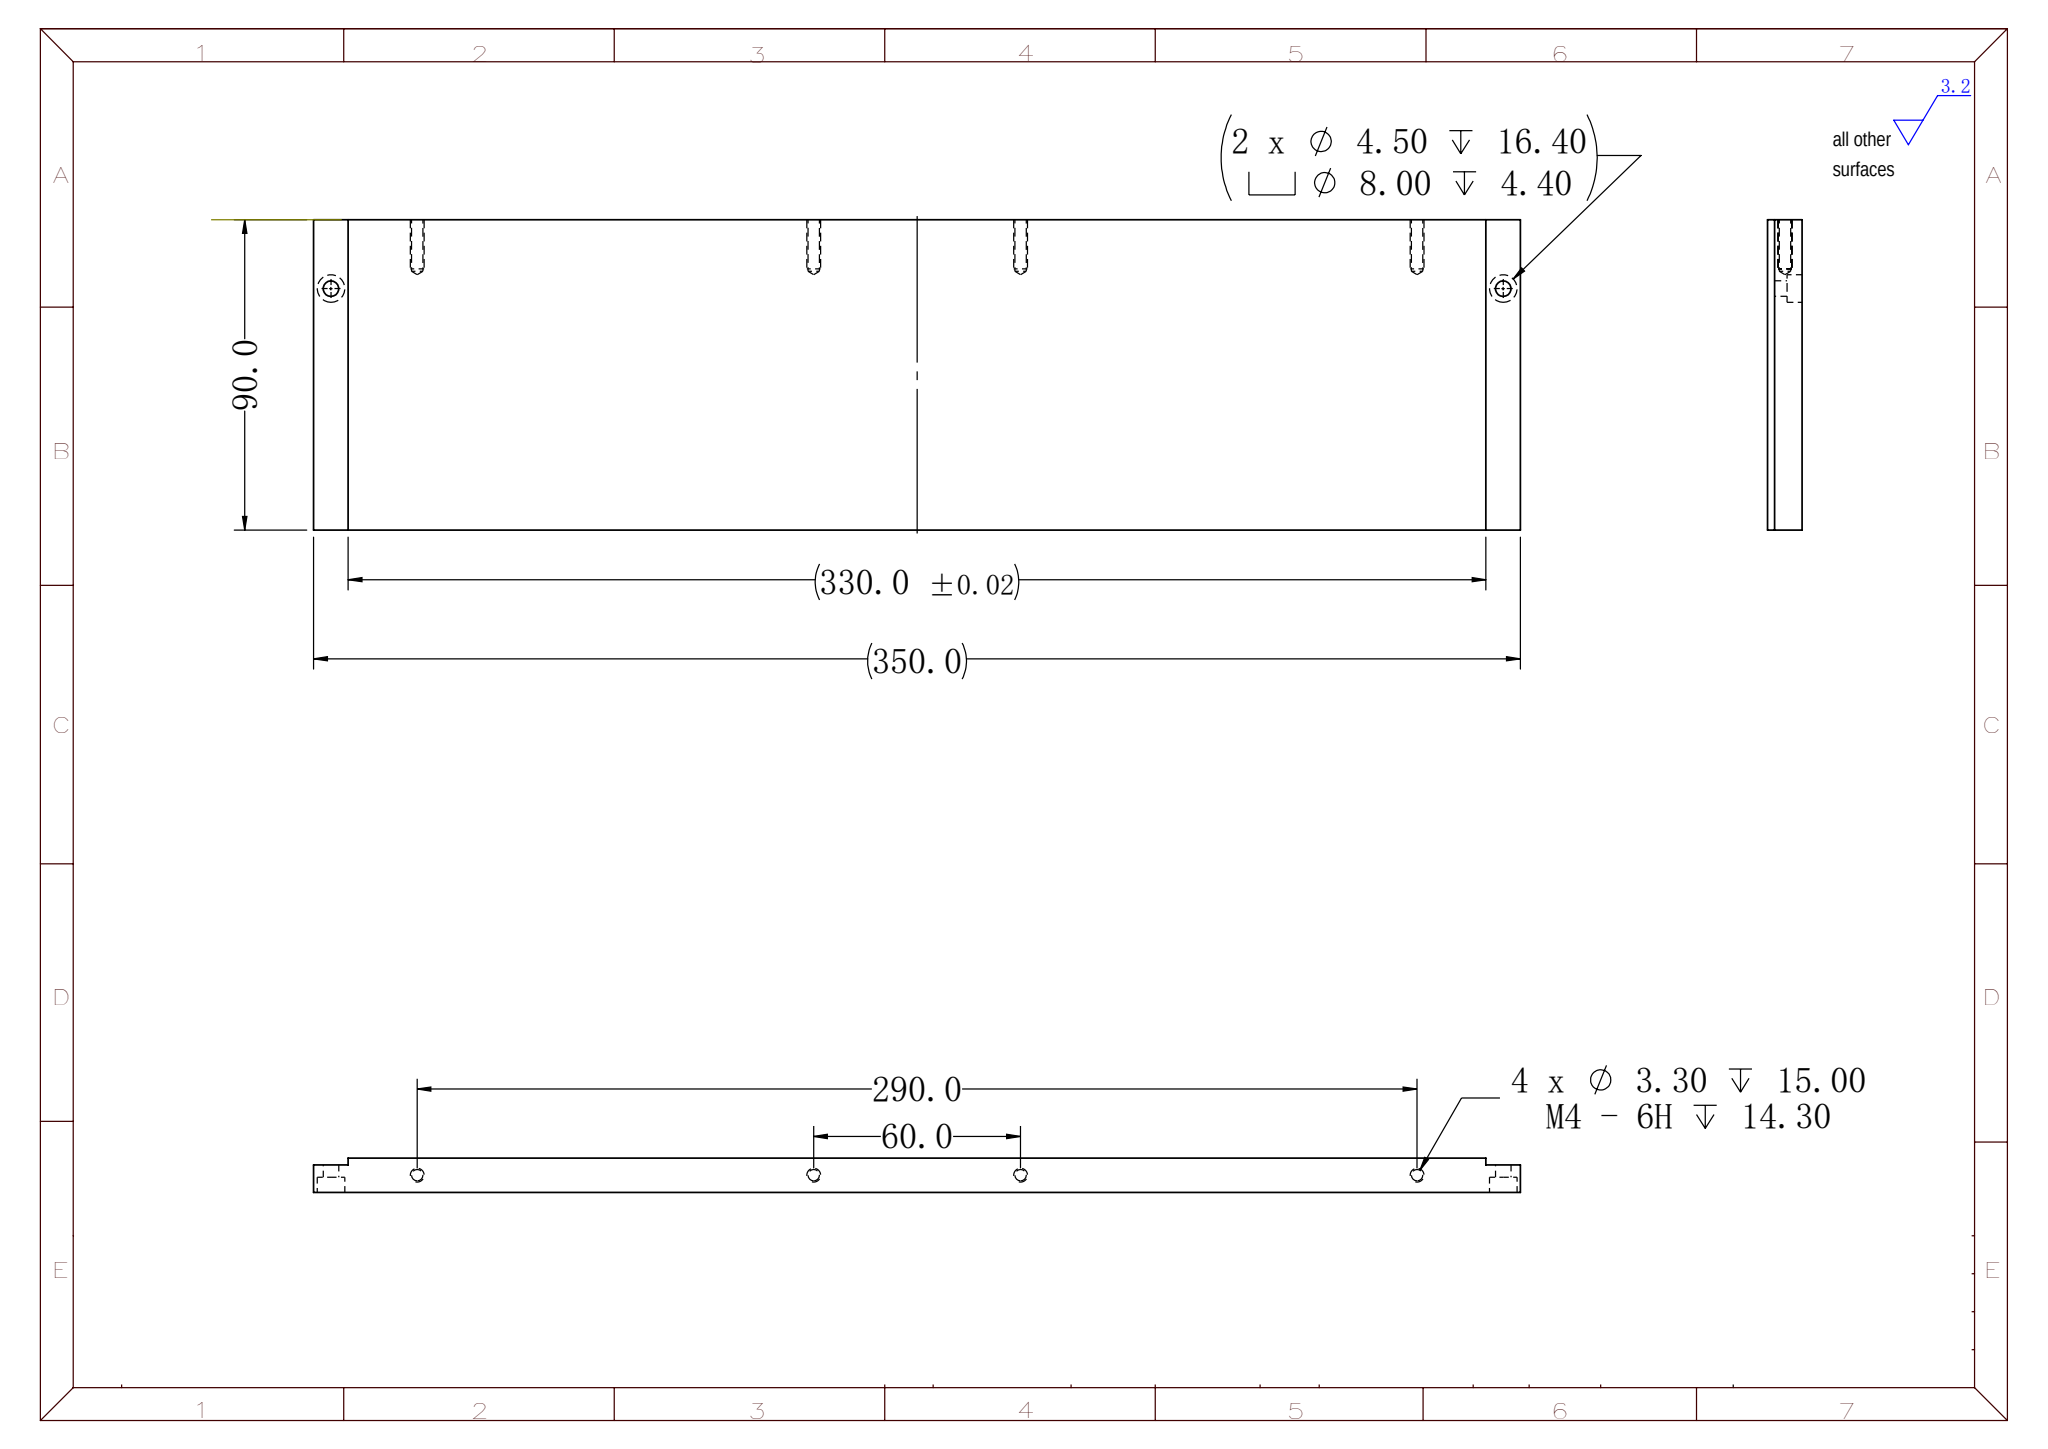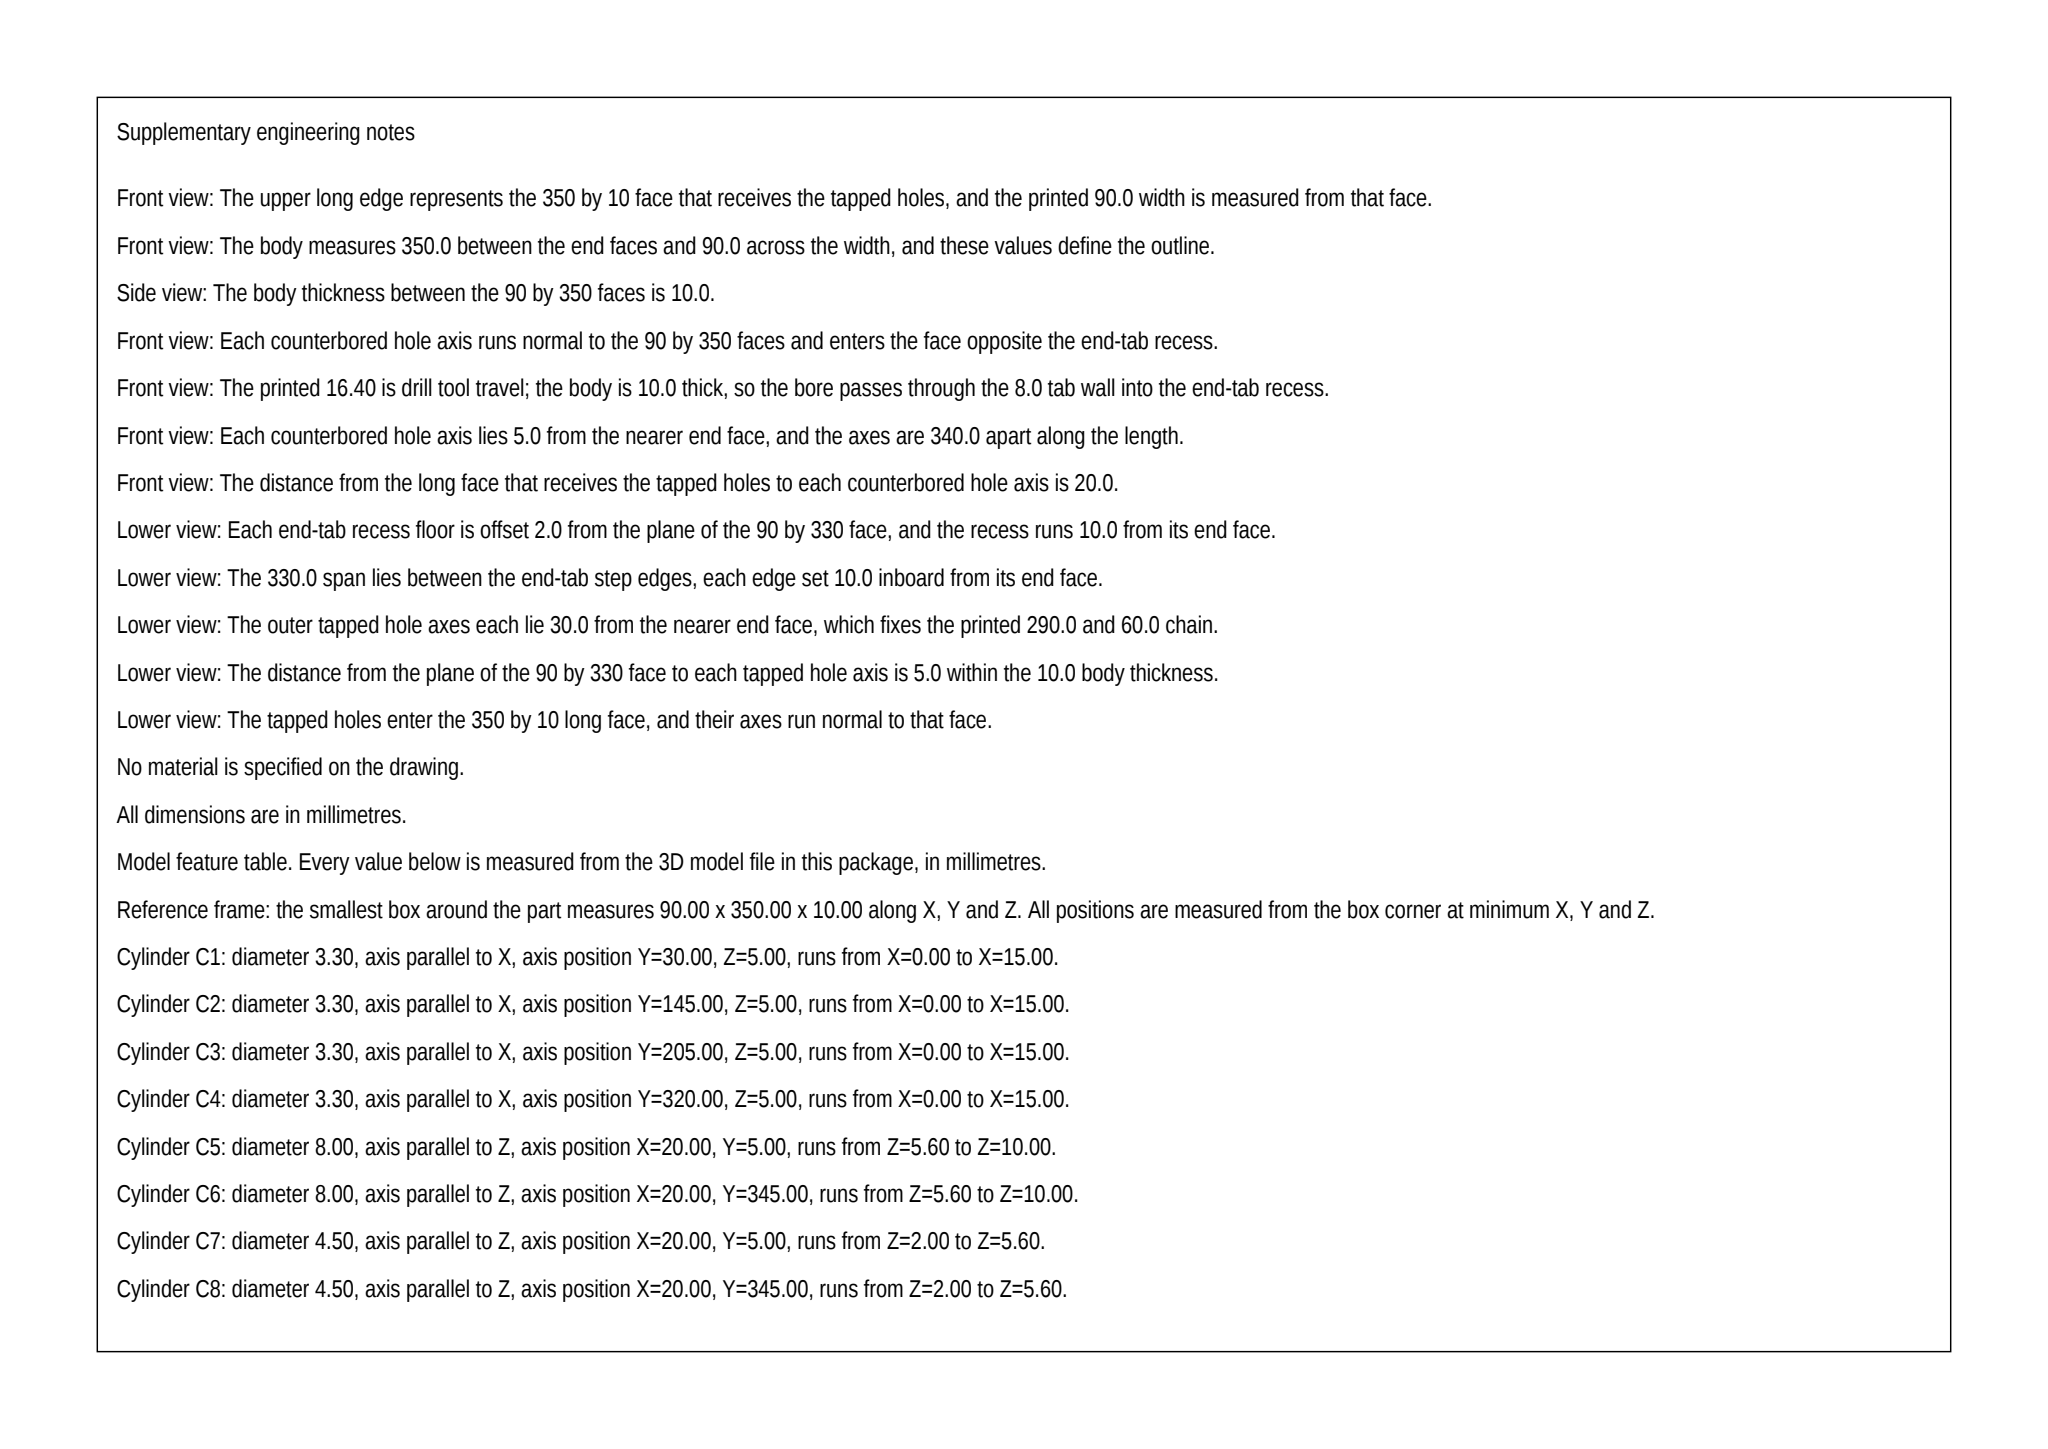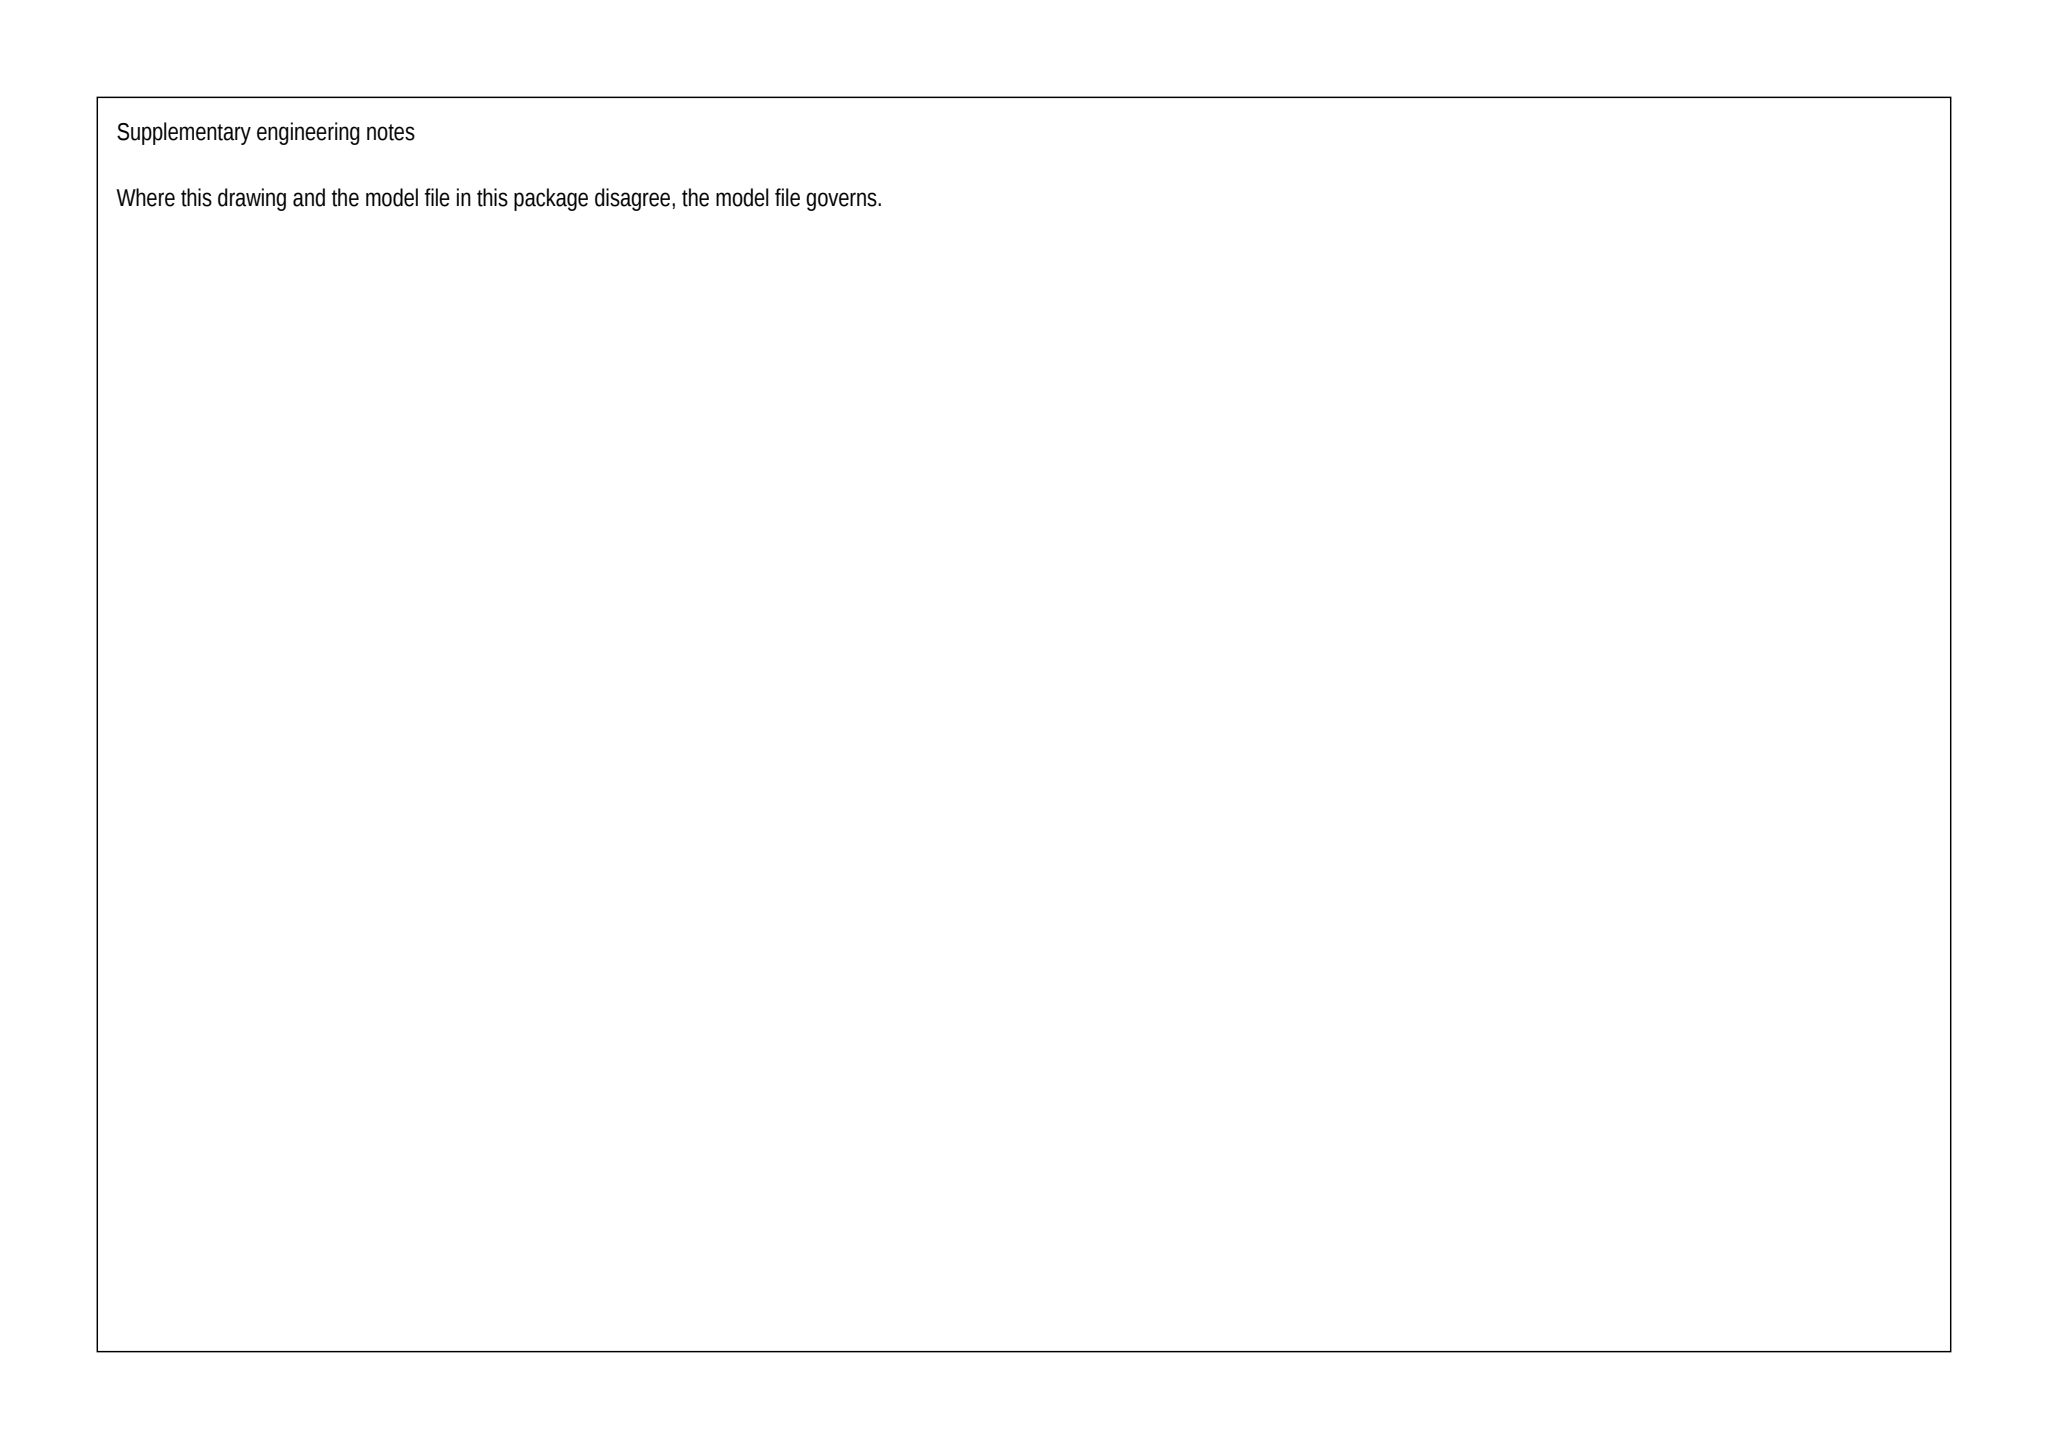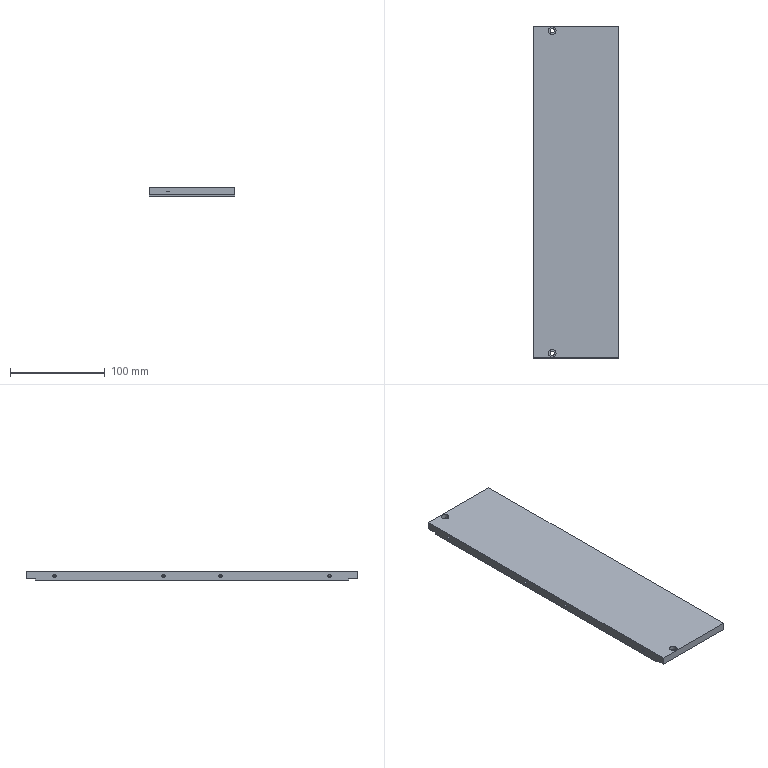Part | SolidWorks | mm | 1 solid | 36 faces | box 90 x 350 x 10 mm | volume 310319 mm3 | cylinder 16 | plane 12 | cone 8 | commonest cylinder face diameters 3.3 x8 8 x4 4.5 x4
Drawing notes:
OVERALL THK 10.0 (SIDE VIEW) | from the solid: bbox_xyz z = 10.0; planes z=0.0 and z=10.0
2X CBORE HOLES: 20.0 FROM TOP EDGE, 5.0 FROM EA END | from the solid: Ø4.5/Ø8.0 axes at (x=20.0, y=5.0) and (x=20.0, y=345.0); bbox y=350.0
4X Ø3.30/M4-6H HOLES ON CL, 5.0 FROM EA FACE (MID-THK) | from the solid: Ø3.3 x-axis holes at z=5.0, thickness 10.0
ALL DIMS IN MM UNLESS OTHERWISE SPECIFIED | from the solid: STEP model units mm; bbox 90.0 x 350.0 x 10.0
STEP EA END: 10 LG x 2.0 DEEP FROM BOTTOM FACE (THK 10 TO 8) | from the solid: z planes at 0, 2.0 (x2) & 10.0; y planes at 10.0 & 340.0 vs bbox 350 long, 10 thk